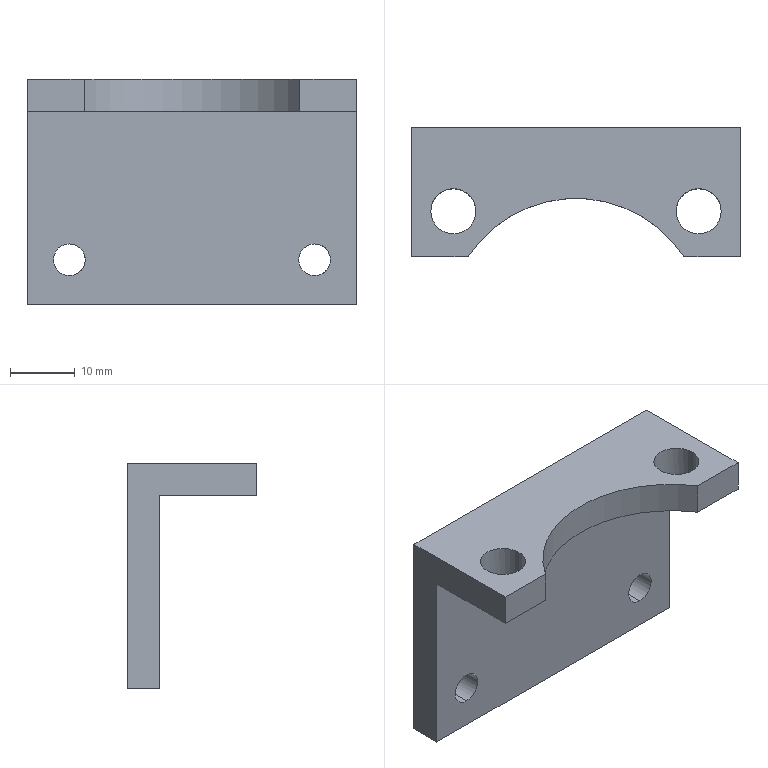CAM job | Mastercam | mm | 13 operations | part box 51 x 20 x 35
1. Contour (Ramp) | 23 - 17 平铣刀
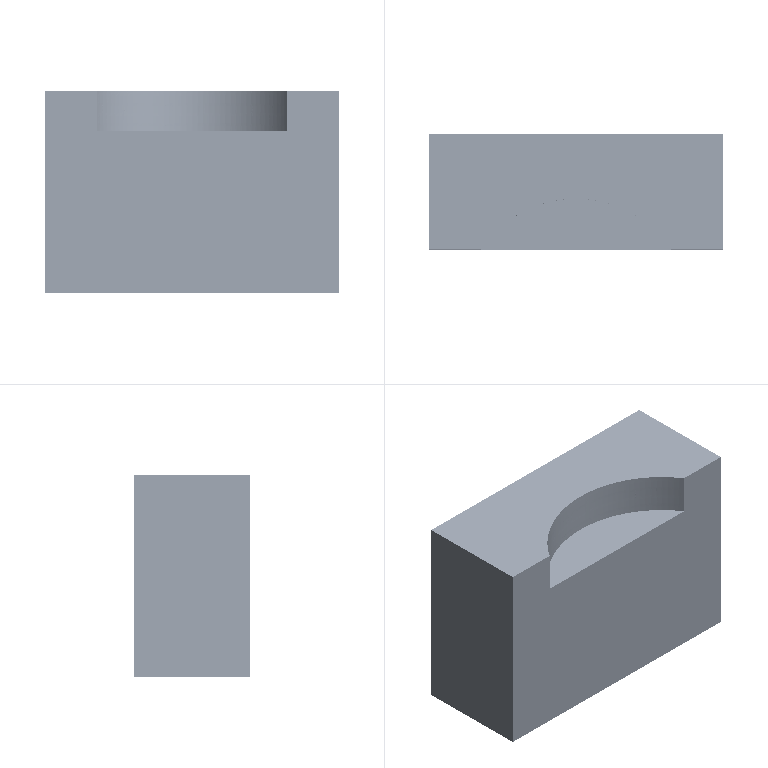2. Contour (2D) | 10 - 10 平铣刀
3. Drill/Counterbore | 2 - 7.94 中心钻
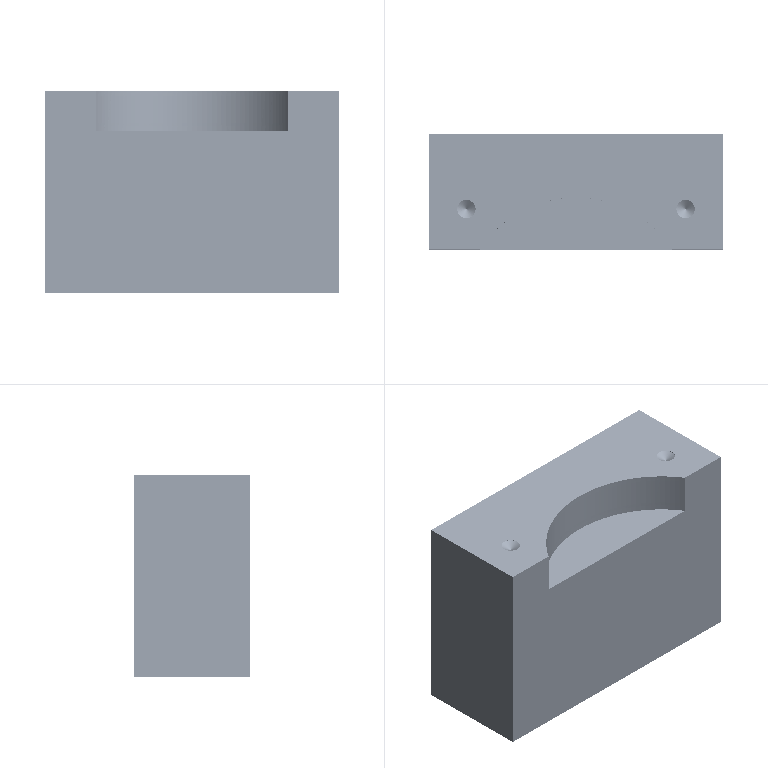4. Peck Drill | 3 - 7 钻头
5. Contour (2D chamfer) | 1 - 6 倒角刀
6. Contour (2D) | 23 - 17 平铣刀
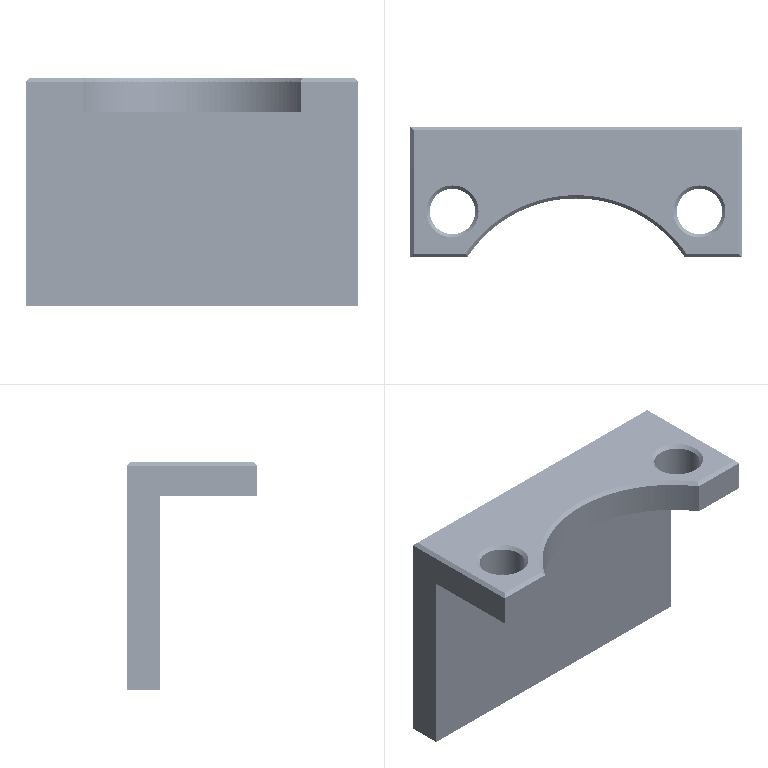7. Drill/Counterbore | 2 - 7.94 中心钻
8. Peck Drill | 4 - 5.1 钻头
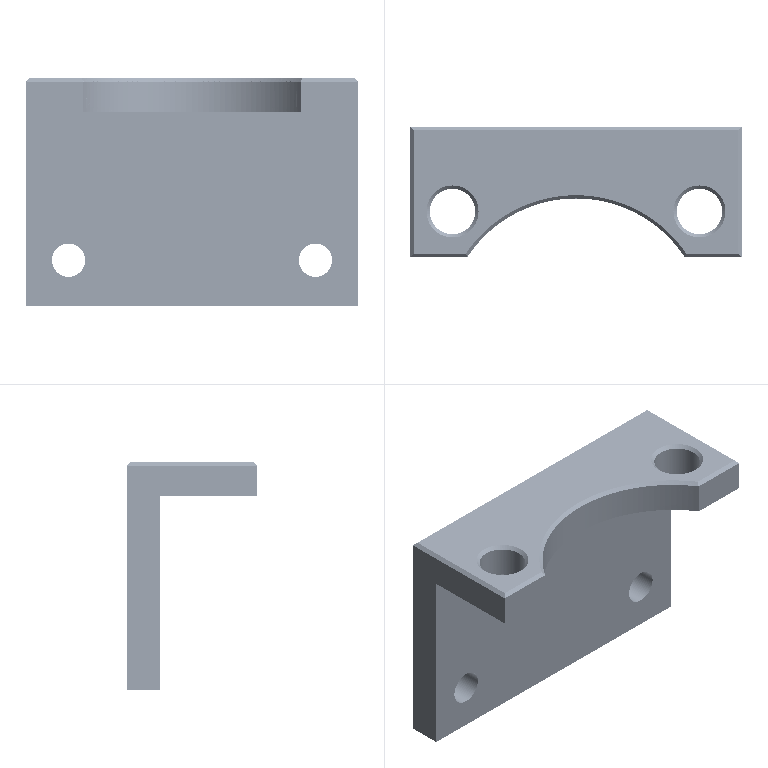9. Contour (2D) | 10 - 10 平铣刀
10. Contour (2D) | 10 - 10 平铣刀
11. Contour (2D chamfer) | 1 - 6 倒角刀
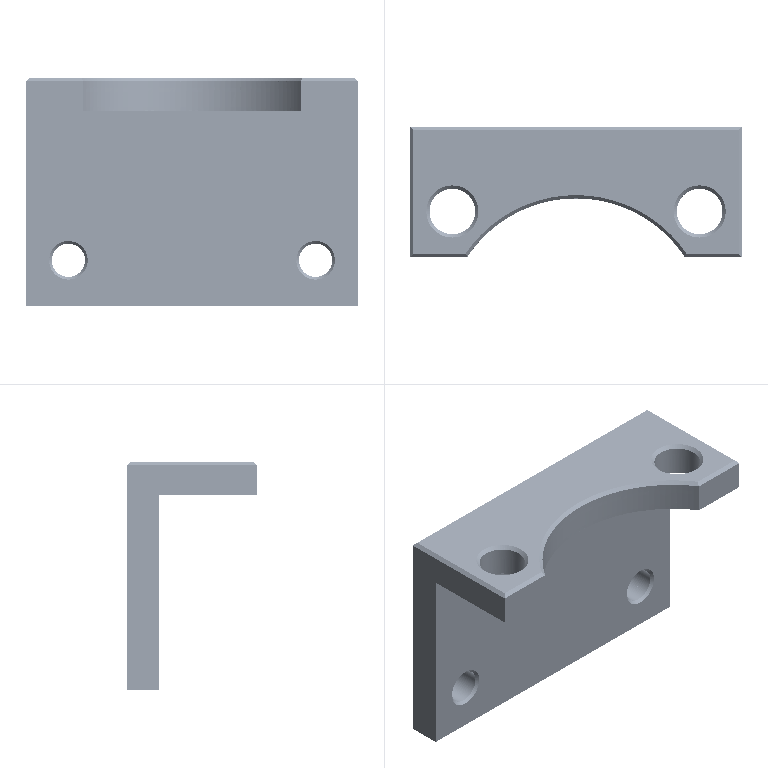12. Contour (2D chamfer) | 1 - 6 倒角刀
13. Deburr 5-axis | 5 - 4 球刀/圆鼻铣刀